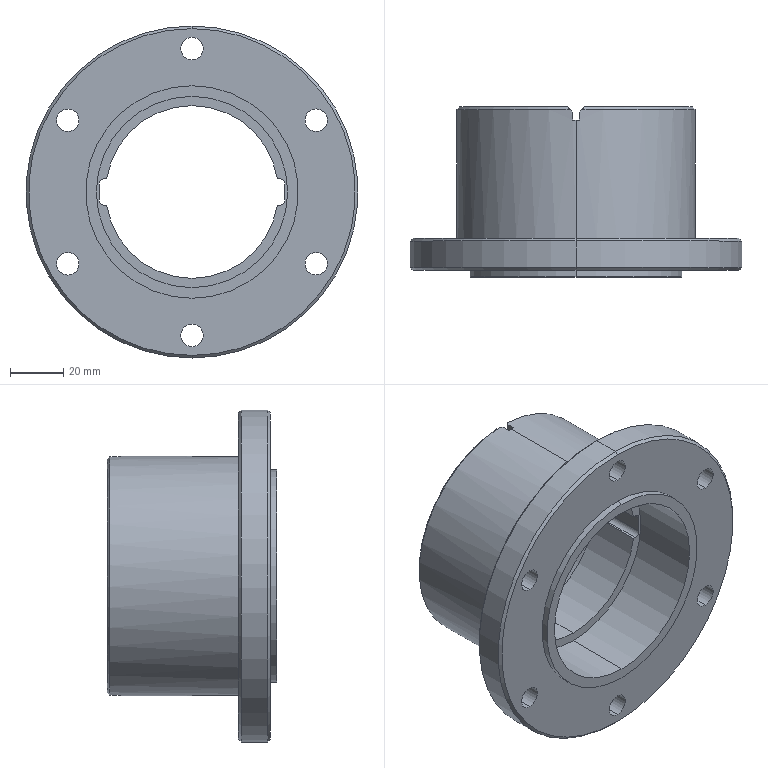Component | SolidWorks | MA060.03.03-03-1 | 1 solid | 58 faces | box 125 x 64 x 125 mm | volume 223683 mm3 | cylinder 29 | plane 23 | cone 6 | commonest cylinder face diameters 8.5 x12 72 x4 4 x4 65 x3 125 x2 90 x2 80 x2 | material 45#
build123d program:
from build123d import *

# Parameters (mm, degrees)
F_8_5_8_5_DIAMETER_HOLE1_D = 8.5
CIRPATTERN1_COUNT          = 6
CHAMFER1_SIZE              = 1
SKETCH4_W                  = 2.5
SKETCH4_H                  = 5
CUT_EXTRUDE1_DEPTH         = 100
CHAMFER2_SIZE              = 2
SKETCH5_W                  = 70
SKETCH5_H                  = 10
CUT_EXTRUDE2_DEPTH         = 100.874
FILLET1_R                  = 2


with BuildPart() as part:
    # Sketch1 → Revolve1 (revolve)
    with BuildSketch(Plane.XY, mode=Mode.PRIVATE) as revolve1_sk:
        Polygon((40, 2.5), (62.5, 2.5), (62.5, 14.5), (45, 14.5), (45, 64), (36, 64), (36, 46.5), (32.5, 46.5), (32.5, 26), (36, 26), (36, 0), (40, 0), align=None)
    revolve(revolve1_sk.sketch.rotate(Axis((0, 0, 0), (0, 1, 0)), 90), axis=Axis((0, 0, 0), (0, 1, 0)))

    # 8.5 _8.5_ Diameter Hole1 (through all)
    with Locations(Plane(origin=(0, 14.5, 0), x_dir=(-1, 0, 0), z_dir=(0, 1, 0))):
        with Locations((0, -54)):
            f_8_5_8_5_diameter_hole1 = Hole(F_8_5_8_5_DIAMETER_HOLE1_D / 2)

    # CirPattern1: 8.5 _8.5_ Diameter Hole1 ×6 about axis
    cirpattern1_axis = Axis((0, 0, 0), (0, 1, 0))
    for i in range(1, CIRPATTERN1_COUNT):
        add(f_8_5_8_5_diameter_hole1.rotate(cirpattern1_axis, i * 360 / CIRPATTERN1_COUNT), mode=Mode.SUBTRACT)

    # Chamfer1
    chamfer1_edges = [part.edges().sort_by_distance(p)[0] for p in [
        (0, 64, 45),
        (0, 2.5, 62.5),
        (0, 14.5, 62.5),
    ]]
    chamfer(chamfer1_edges, length=CHAMFER1_SIZE)

    # Sketch4 → Cut-Extrude1 (cut, symmetric)
    with BuildSketch(Plane.XY):
        with Locations((0, 61.5)):
            Rectangle(SKETCH4_W, SKETCH4_H)
    extrude(amount=CUT_EXTRUDE1_DEPTH, both=True, mode=Mode.SUBTRACT)

    # Chamfer2
    chamfer2_edges = [part.edges().sort_by_distance(p)[0] for p in [
        (1.25, 64, 39.98),
        (1.25, 64, -39.98),
        (-1.25, 64, -39.98),
        (-1.25, 64, 39.98),
    ]]
    chamfer(chamfer2_edges, length=CHAMFER2_SIZE)

    # Sketch5 → Cut-Extrude2 (cut, through all)
    with BuildSketch(Plane(origin=(0, 46.5, 0), x_dir=(1, 0, 0), z_dir=(0, 1, 0))):
        Rectangle(SKETCH5_W, SKETCH5_H)
    extrude(amount=-CUT_EXTRUDE2_DEPTH, mode=Mode.SUBTRACT)

    # Fillet1
    fillet1_edges = [part.edges().sort_by_distance(p)[0] for p in [
        (35, 36.25, -5),
        (35, 36.25, 5),
        (-35, 36.25, 5),
        (-35, 36.25, -5),
    ]]
    fillet(fillet1_edges, radius=FILLET1_R)


solid = part.part